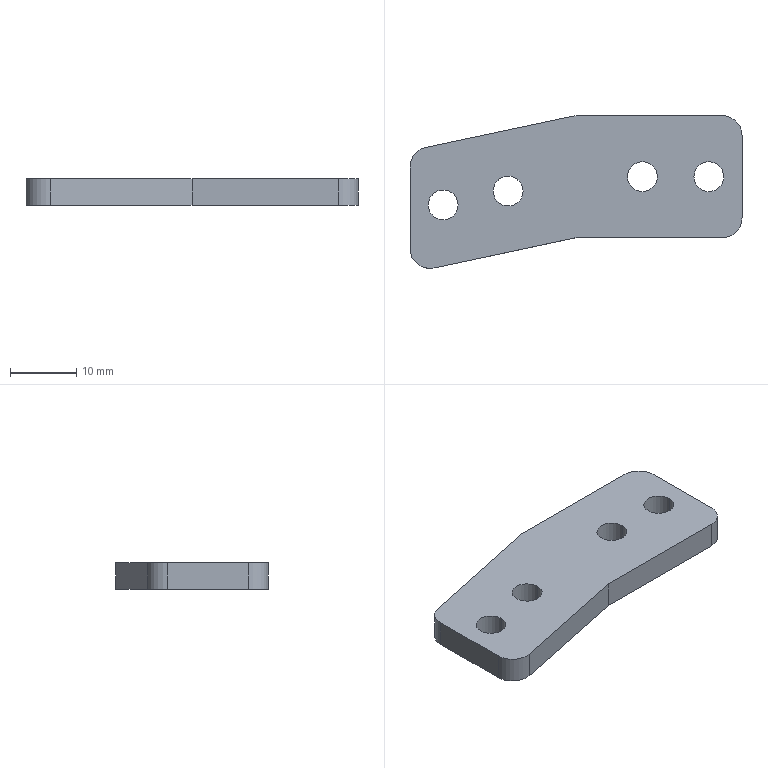Component | SolidWorks | 3RearBaffleConnectionPlate9.26-1 | 1 solid | 20 faces | box 50 x 23.01 x 4 mm | volume 3393 mm3 | cylinder 12 | plane 8 | commonest cylinder face diameters 4.5 x8 6 x4 | material AISI 1045 Steel, Cold Drawn
build123d program:
from build123d import *

# Parameters (mm, degrees)
BOSS_EXTRUDE1_DEPTH = 4
FILLET1_R           = 3
SKETCH3_R           = 2.25
CUT_EXTRUDE1_DEPTH  = 32.299


with BuildPart() as part:
    # Sketch1 → Boss-Extrude1 (new body)
    with BuildSketch(Plane.XY):
        Polygon((0, 18.402), (25, 18.402), (25, 0), (0, 0), (-25, -5.314), (-25, 13.088), align=None)
    extrude(amount=BOSS_EXTRUDE1_DEPTH)

    # Fillet1
    fillet1_edges = [part.edges().sort_by_distance(p)[0] for p in [
        (-25, -5.314, 2),
        (-25, 13.088, 2),
        (25, 18.402, 2),
        (25, 0, 2),
    ]]
    fillet(fillet1_edges, radius=FILLET1_R)

    # Sketch3 → Cut-Extrude1 (cut, through all)
    with BuildSketch(Plane.XY.offset(4)):
        with Locations((20, 9.201)):
            Circle(SKETCH3_R)
        with Locations((10, 9.201)):
            Circle(SKETCH3_R)
        with Locations((-20, 4.95)):
            Circle(SKETCH3_R)
        with Locations((-10.219, 7.029)):
            Circle(SKETCH3_R)
    extrude(amount=-CUT_EXTRUDE1_DEPTH, mode=Mode.SUBTRACT)


solid = part.part

# Placed as in the assembly
solid = solid.moved(Location((395.259, 105.763, 17.75), (0, 0, 0)))